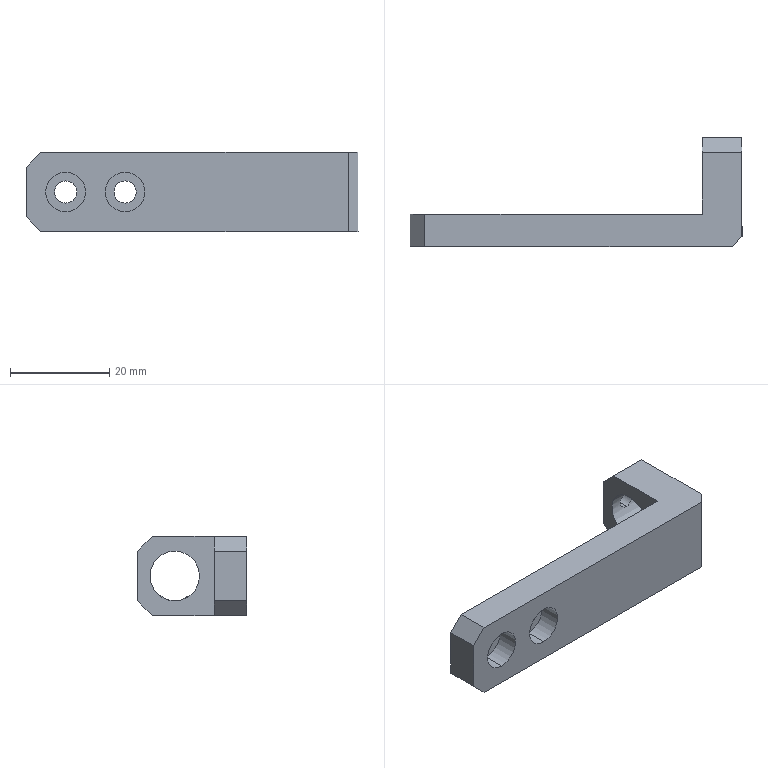Component | SolidWorks | 016WindShieldHolder-1 | 1 solid | 29 faces | box 67 x 22 x 16 mm | volume 7604 mm3 | plane 15 | cylinder 14 | commonest cylinder face diameters 3.3 x4 8 x4 4.5 x4 10 x2
build123d program:
from build123d import *

# Parameters (mm, degrees)
SKETCH1_W                                           = 67
SKETCH1_H                                           = 22
BOSS_EXTRUDE1_DEPTH                                 = 16
SKETCH2_W                                           = 59
SKETCH2_H                                           = 15.5
CUT_EXTRUDE1_DEPTH                                  = 73.312
M4_HEX_SOCKET_HEAD_CAP_SCREW_POST_HOLE1_D           = 4.5
M4_HEX_SOCKET_HEAD_CAP_SCREW_POST_HOLE1_CBORE_D     = 8
M4_HEX_SOCKET_HEAD_CAP_SCREW_POST_HOLE1_CBORE_DEPTH = 4.4
SKETCH5_R                                           = 5
CUT_EXTRUDE2_DEPTH                                  = 73.312
CHAMFER1_SIZE                                       = 3
M4_TAPPED_HOLE1_D                                   = 3.3
M4_TAPPED_HOLE1_DEPTH                               = 6.1
M4_TAPPED_HOLE1_TIP                                 = 0.9914
M4_TAPPED_HOLE2_D                                   = 3.3
M4_TAPPED_HOLE2_DEPTH                               = 6.1
M4_TAPPED_HOLE2_TIP                                 = 0.9914
CHAMFER2_SIZE                                       = 2


with BuildPart() as part:
    # Sketch1 → Boss-Extrude1 (new body)
    with BuildSketch(Plane.XY):
        with Locations((33.5, 11)):
            Rectangle(SKETCH1_W, SKETCH1_H)
    extrude(amount=BOSS_EXTRUDE1_DEPTH)

    # Sketch2 → Cut-Extrude1 (cut, through all)
    with BuildSketch(Plane.XY.offset(16)):
        with Locations((37.5, 14.25)):
            Rectangle(SKETCH2_W, SKETCH2_H)
    extrude(amount=-CUT_EXTRUDE1_DEPTH, mode=Mode.SUBTRACT)

    # M4 Hex Socket Head Cap Screw Post Hole1 (through all)
    with Locations(Plane(origin=(0, 0, 0), x_dir=(-1, 0, 0), z_dir=(0, -1, 0))):
        with Locations((-59, -8), (-47, -8)):
            CounterBoreHole(M4_HEX_SOCKET_HEAD_CAP_SCREW_POST_HOLE1_D / 2, M4_HEX_SOCKET_HEAD_CAP_SCREW_POST_HOLE1_CBORE_D / 2, M4_HEX_SOCKET_HEAD_CAP_SCREW_POST_HOLE1_CBORE_DEPTH)

    # Sketch5 → Cut-Extrude2 (cut, through all)
    with BuildSketch(Plane.ZY):
        with Locations((8, 14.5)):
            Circle(SKETCH5_R)
    extrude(amount=-CUT_EXTRUDE2_DEPTH, mode=Mode.SUBTRACT)

    # Chamfer1
    chamfer1_edges = [part.edges().sort_by_distance(p)[0] for p in [
        (67, 3.25, 16),
        (4, 22, 0),
        (4, 22, 16),
        (67, 3.25, 0),
    ]]
    chamfer(chamfer1_edges, length=CHAMFER1_SIZE)

    # M4 Tapped Hole1
    with Locations(Plane(origin=(0, 22, 0), x_dir=(1, 0, 0), z_dir=(0, 1, 0))):
        with Locations((4, -8)):
            Hole(M4_TAPPED_HOLE1_D / 2, depth=M4_TAPPED_HOLE1_DEPTH)
            with Locations((0, 0, -(M4_TAPPED_HOLE1_DEPTH + M4_TAPPED_HOLE1_TIP / 2))):  # 118° drill point
                Cone(0, M4_TAPPED_HOLE1_D / 2, M4_TAPPED_HOLE1_TIP, mode=Mode.SUBTRACT)

    # M4 Tapped Hole2
    with Locations(Plane.XY.offset(16)):
        with Locations((4, 14.5)):
            Hole(M4_TAPPED_HOLE2_D / 2, depth=M4_TAPPED_HOLE2_DEPTH)
            with Locations((0, 0, -(M4_TAPPED_HOLE2_DEPTH + M4_TAPPED_HOLE2_TIP / 2))):  # 118° drill point
                Cone(0, M4_TAPPED_HOLE2_D / 2, M4_TAPPED_HOLE2_TIP, mode=Mode.SUBTRACT)

    # Chamfer2
    chamfer2_edges = [part.edges().sort_by_distance(p)[0] for p in [
        (0, 0, 8),
    ]]
    chamfer(chamfer2_edges, length=CHAMFER2_SIZE)


solid = part.part

# Placed as in the assembly
solid = solid.moved(Location((86.76, 60.179, 19), (-180, 0, 180)))
STEP:
#1=COLOUR_RGB('',0.7922,0.8196,0.9333);
#2=FILL_AREA_STYLE_COLOUR('',#1);
#3=FILL_AREA_STYLE('',(#2));
#4=SURFACE_STYLE_FILL_AREA(#3);
#5=SURFACE_SIDE_STYLE('',(#4));
#6=SURFACE_STYLE_USAGE(.BOTH.,#5);
#7=PRESENTATION_STYLE_ASSIGNMENT((#6));
#8=CARTESIAN_POINT('',(3.323,2.94,0.2362));
#9=VERTEX_POINT('',#8);
#10=CARTESIAN_POINT('',(3.193,2.94,0.2362));
#11=VERTEX_POINT('',#10);
#12=CARTESIAN_POINT('',(3.323,2.94,0.2362));
#13=CARTESIAN_POINT('',(3.323,2.932,0.2362));
#14=CARTESIAN_POINT('',(3.321,2.923,0.2368));
#15=CARTESIAN_POINT('',(3.317,2.911,0.2383));
#16=CARTESIAN_POINT('',(3.315,2.907,0.2389));
#17=CARTESIAN_POINT('',(3.31,2.9,0.2402));
#18=CARTESIAN_POINT('',(3.307,2.897,0.2409));
#19=CARTESIAN_POINT('',(3.298,2.888,0.2431));
#20=CARTESIAN_POINT('',(3.291,2.883,0.2445));
#21=CARTESIAN_POINT('',(3.279,2.878,0.2461));
#22=CARTESIAN_POINT('',(3.275,2.877,0.2465));
#23=CARTESIAN_POINT('',(3.267,2.876,0.2471));
#24=CARTESIAN_POINT('',(3.263,2.875,0.2472));
#25=CARTESIAN_POINT('',(3.254,2.875,0.2472));
#26=CARTESIAN_POINT('',(3.25,2.876,0.2471));
#27=CARTESIAN_POINT('',(3.241,2.877,0.2465));
#28=CARTESIAN_POINT('',(3.237,2.879,0.2461));
#29=CARTESIAN_POINT('',(3.225,2.883,0.2445));
#30=CARTESIAN_POINT('',(3.218,2.888,0.2431));
#31=CARTESIAN_POINT('',(3.209,2.897,0.2409));
#32=CARTESIAN_POINT('',(3.207,2.9,0.2402));
#33=CARTESIAN_POINT('',(3.202,2.907,0.2389));
#34=CARTESIAN_POINT('',(3.2,2.911,0.2383));
#35=CARTESIAN_POINT('',(3.197,2.919,0.2373));
#36=CARTESIAN_POINT('',(3.195,2.923,0.2369));
#37=CARTESIAN_POINT('',(3.194,2.932,0.2364));
#38=CARTESIAN_POINT('',(3.193,2.936,0.2362));
#39=CARTESIAN_POINT('',(3.193,2.94,0.2362));
#40=B_SPLINE_CURVE_WITH_KNOTS('',3,(#12,#13,#14,#15,#16,#17,#18,#19,#20,#21,#22,#23,#24,#25,#26,#27,#28,#29,#30,#31,#32,#33,#34,#35,#36,#37,#38,#39),.UNSPECIFIED.,.F.,.F.,(4,2,2,2,2,2,2,2,2,2,2,2,2,4),(0.005195,0.005845,0.006169,0.006494,0.007143,0.007468,0.007792,0.008117,0.008442,0.009091,0.009415,0.00974,0.01006,0.01039),.UNSPECIFIED.);
#41=EDGE_CURVE('',#9,#11,#40,.T.);
#42=ORIENTED_EDGE('',*,*,#41,.F.);
#43=CARTESIAN_POINT('',(3.323,2.94,0.1181));
#44=VERTEX_POINT('',#43);
#45=CARTESIAN_POINT('',(3.323,2.94,0.1181));
#46=DIRECTION('',(0.,0.,-1.));
#47=VECTOR('',#46,39.37);
#48=LINE('',#45,#47);
#49=EDGE_CURVE('',#9,#44,#48,.T.);
#50=ORIENTED_EDGE('',*,*,#49,.T.);
#51=CARTESIAN_POINT('',(3.193,2.94,0.1181));
#52=VERTEX_POINT('',#51);
#53=CARTESIAN_POINT('',(3.258,2.94,0.1181));
#54=DIRECTION('',(0.,0.,-1.));
#55=DIRECTION('',(-1.,0.,-0.));
#56=AXIS2_PLACEMENT_3D('',#53,#54,#55);
#57=CIRCLE('',#56,0.06496);
#58=EDGE_CURVE('',#44,#52,#57,.T.);
#59=ORIENTED_EDGE('',*,*,#58,.T.);
#60=CARTESIAN_POINT('',(3.193,2.94,0.1181));
#61=DIRECTION('',(0.,0.,-1.));
#62=VECTOR('',#61,39.37);
#63=LINE('',#60,#62);
#64=EDGE_CURVE('',#11,#52,#63,.T.);
#65=ORIENTED_EDGE('',*,*,#64,.F.);
#66=EDGE_LOOP('',(#42,#50,#59,#65));
#67=FACE_OUTER_BOUND('',#66,.T.);
#68=CARTESIAN_POINT('',(3.258,2.94,0.1181));
#69=DIRECTION('',(0.,0.,-1.));
#70=DIRECTION('',(-1.,0.,-0.));
#71=AXIS2_PLACEMENT_3D('',#68,#69,#70);
#72=CYLINDRICAL_SURFACE('',#71,0.06496);
#73=ADVANCED_FACE('',(#67),#72,.F.);
#74=CARTESIAN_POINT('',(3.258,3.126,0.498));
#75=VERTEX_POINT('',#74);
#76=CARTESIAN_POINT('',(3.258,3.126,0.3681));
#77=VERTEX_POINT('',#76);
#78=CARTESIAN_POINT('',(3.258,3.126,0.498));
#79=CARTESIAN_POINT('',(3.267,3.126,0.498));
#80=CARTESIAN_POINT('',(3.275,3.127,0.4963));
#81=CARTESIAN_POINT('',(3.287,3.128,0.4914));
#82=CARTESIAN_POINT('',(3.291,3.129,0.4894));
#83=CARTESIAN_POINT('',(3.298,3.13,0.4847));
#84=CARTESIAN_POINT('',(3.301,3.131,0.482));
#85=CARTESIAN_POINT('',(3.31,3.133,0.473));
#86=CARTESIAN_POINT('',(3.315,3.134,0.4659));
#87=CARTESIAN_POINT('',(3.32,3.136,0.4541));
#88=CARTESIAN_POINT('',(3.321,3.136,0.45));
#89=CARTESIAN_POINT('',(3.323,3.137,0.4417));
#90=CARTESIAN_POINT('',(3.323,3.137,0.4373));
#91=CARTESIAN_POINT('',(3.323,3.137,0.4288));
#92=CARTESIAN_POINT('',(3.323,3.137,0.4245));
#93=CARTESIAN_POINT('',(3.321,3.136,0.4162));
#94=CARTESIAN_POINT('',(3.32,3.136,0.412));
#95=CARTESIAN_POINT('',(3.315,3.134,0.4003));
#96=CARTESIAN_POINT('',(3.31,3.133,0.3931));
#97=CARTESIAN_POINT('',(3.301,3.131,0.3842));
#98=CARTESIAN_POINT('',(3.298,3.13,0.3814));
#99=CARTESIAN_POINT('',(3.291,3.129,0.3767));
#100=CARTESIAN_POINT('',(3.287,3.128,0.3747));
#101=CARTESIAN_POINT('',(3.279,3.127,0.3715));
#102=CARTESIAN_POINT('',(3.275,3.127,0.3702));
#103=CARTESIAN_POINT('',(3.267,3.126,0.3685));
#104=CARTESIAN_POINT('',(3.263,3.126,0.3681));
#105=CARTESIAN_POINT('',(3.258,3.126,0.3681));
#106=B_SPLINE_CURVE_WITH_KNOTS('',3,(#78,#79,#80,#81,#82,#83,#84,#85,#86,#87,#88,#89,#90,#91,#92,#93,#94,#95,#96,#97,#98,#99,#100,#101,#102,#103,#104,#105),.UNSPECIFIED.,.F.,.F.,(4,2,2,2,2,2,2,2,2,2,2,2,2,4),(0.005195,0.005844,0.006169,0.006494,0.007143,0.007467,0.007792,0.008117,0.008441,0.009091,0.009415,0.00974,0.01006,0.01039),.UNSPECIFIED.);
#107=EDGE_CURVE('',#75,#77,#106,.T.);
#108=ORIENTED_EDGE('',*,*,#107,.F.);
#109=CARTESIAN_POINT('',(3.258,3.235,0.498));
#110=VERTEX_POINT('',#109);
#111=CARTESIAN_POINT('',(3.258,3.235,0.498));
#112=DIRECTION('',(-0.,1.,0.));
#113=VECTOR('',#112,39.37);
#114=LINE('',#111,#113);
#115=EDGE_CURVE('',#75,#110,#114,.T.);
#116=ORIENTED_EDGE('',*,*,#115,.T.);
#117=CARTESIAN_POINT('',(3.258,3.235,0.3681));
#118=VERTEX_POINT('',#117);
#119=CARTESIAN_POINT('',(3.258,3.235,0.4331));
#120=DIRECTION('',(-0.,1.,0.));
#121=DIRECTION('',(0.,0.,-1.));
#122=AXIS2_PLACEMENT_3D('',#119,#120,#121);
#123=CIRCLE('',#122,0.06496);
#124=EDGE_CURVE('',#110,#118,#123,.T.);
#125=ORIENTED_EDGE('',*,*,#124,.T.);
#126=CARTESIAN_POINT('',(3.258,3.235,0.3681));
#127=DIRECTION('',(-0.,1.,0.));
#128=VECTOR('',#127,39.37);
#129=LINE('',#126,#128);
#130=EDGE_CURVE('',#77,#118,#129,.T.);
#131=ORIENTED_EDGE('',*,*,#130,.F.);
#132=EDGE_LOOP('',(#108,#116,#125,#131));
#133=FACE_OUTER_BOUND('',#132,.T.);
#134=CARTESIAN_POINT('',(3.258,3.235,0.4331));
#135=DIRECTION('',(-0.,1.,0.));
#136=DIRECTION('',(0.,0.,-1.));
#137=AXIS2_PLACEMENT_3D('',#134,#135,#136);
#138=CYLINDRICAL_SURFACE('',#137,0.06496);
#139=ADVANCED_FACE('',(#133),#138,.F.);
#140=CARTESIAN_POINT('',(3.101,2.94,0.6299));
#141=VERTEX_POINT('',#140);
#142=CARTESIAN_POINT('',(3.101,2.94,0.2362));
#143=VERTEX_POINT('',#142);
#144=CARTESIAN_POINT('',(3.101,2.94,0.4331));
#145=DIRECTION('',(1.,0.,0.));
#146=DIRECTION('',(0.,0.,-1.));
#147=AXIS2_PLACEMENT_3D('',#144,#145,#146);
#148=CIRCLE('',#147,0.1969);
#149=EDGE_CURVE('',#141,#143,#148,.T.);
#150=ORIENTED_EDGE('',*,*,#149,.F.);
#151=CARTESIAN_POINT('',(3.416,2.94,0.6299));
#152=VERTEX_POINT('',#151);
#153=CARTESIAN_POINT('',(0.7779,2.94,0.6299));
#154=DIRECTION('',(1.,0.,0.));
#155=VECTOR('',#154,39.37);
#156=LINE('',#153,#155);
#157=EDGE_CURVE('',#141,#152,#156,.T.);
#158=ORIENTED_EDGE('',*,*,#157,.T.);
#159=CARTESIAN_POINT('',(3.416,2.94,0.2362));
#160=VERTEX_POINT('',#159);
#161=CARTESIAN_POINT('',(3.416,2.94,0.4331));
#162=DIRECTION('',(1.,0.,0.));
#163=DIRECTION('',(0.,0.,-1.));
#164=AXIS2_PLACEMENT_3D('',#161,#162,#163);
#165=CIRCLE('',#164,0.1969);
#166=EDGE_CURVE('',#152,#160,#165,.T.);
#167=ORIENTED_EDGE('',*,*,#166,.T.);
#168=CARTESIAN_POINT('',(0.7779,2.94,0.2362));
#169=DIRECTION('',(1.,0.,0.));
#170=VECTOR('',#169,39.37);
#171=LINE('',#168,#170);
#172=EDGE_CURVE('',#9,#160,#171,.T.);
#173=ORIENTED_EDGE('',*,*,#172,.F.);
#174=ORIENTED_EDGE('',*,*,#41,.T.);
#175=CARTESIAN_POINT('',(0.7779,2.94,0.2362));
#176=DIRECTION('',(1.,0.,0.));
#177=VECTOR('',#176,39.37);
#178=LINE('',#175,#177);
#179=EDGE_CURVE('',#143,#11,#178,.T.);
#180=ORIENTED_EDGE('',*,*,#179,.F.);
#181=EDGE_LOOP('',(#150,#158,#167,#173,#174,#180));
#182=FACE_OUTER_BOUND('',#181,.T.);
#183=CARTESIAN_POINT('',(0.7779,2.94,0.4331));
#184=DIRECTION('',(1.,0.,0.));
#185=DIRECTION('',(0.,0.,-1.));
#186=AXIS2_PLACEMENT_3D('',#183,#184,#185);
#187=CYLINDRICAL_SURFACE('',#186,0.1969);
#188=ADVANCED_FACE('',(#182),#187,.F.);
#189=CARTESIAN_POINT('',(1.093,2.542,0.2756));
#190=VERTEX_POINT('',#189);
#191=CARTESIAN_POINT('',(1.093,2.542,0.5906));
#192=VERTEX_POINT('',#191);
#193=CARTESIAN_POINT('',(1.093,2.542,0.4331));
#194=DIRECTION('',(0.,-1.,-0.));
#195=DIRECTION('',(-0.,0.,1.));
#196=AXIS2_PLACEMENT_3D('',#193,#194,#195);
#197=CIRCLE('',#196,0.1575);
#198=EDGE_CURVE('',#190,#192,#197,.T.);
#199=ORIENTED_EDGE('',*,*,#198,.F.);
#200=CARTESIAN_POINT('',(1.093,2.369,0.2756));
#201=VERTEX_POINT('',#200);
#202=CARTESIAN_POINT('',(1.093,2.369,0.2756));
#203=DIRECTION('',(0.,-1.,-0.));
#204=VECTOR('',#203,39.37);
#205=LINE('',#202,#204);
#206=EDGE_CURVE('',#190,#201,#205,.T.);
#207=ORIENTED_EDGE('',*,*,#206,.T.);
#208=CARTESIAN_POINT('',(1.093,2.369,0.5906));
#209=VERTEX_POINT('',#208);
#210=CARTESIAN_POINT('',(1.093,2.369,0.4331));
#211=DIRECTION('',(0.,-1.,-0.));
#212=DIRECTION('',(-0.,0.,1.));
#213=AXIS2_PLACEMENT_3D('',#210,#211,#212);
#214=CIRCLE('',#213,0.1575);
#215=EDGE_CURVE('',#201,#209,#214,.T.);
#216=ORIENTED_EDGE('',*,*,#215,.T.);
#217=CARTESIAN_POINT('',(1.093,2.369,0.5906));
#218=DIRECTION('',(0.,-1.,-0.));
#219=VECTOR('',#218,39.37);
#220=LINE('',#217,#219);
#221=EDGE_CURVE('',#192,#209,#220,.T.);
#222=ORIENTED_EDGE('',*,*,#221,.F.);
#223=EDGE_LOOP('',(#199,#207,#216,#222));
#224=FACE_OUTER_BOUND('',#223,.T.);
#225=CARTESIAN_POINT('',(1.093,2.369,0.4331));
#226=DIRECTION('',(0.,-1.,-0.));
#227=DIRECTION('',(-0.,0.,1.));
#228=AXIS2_PLACEMENT_3D('',#225,#226,#227);
#229=CYLINDRICAL_SURFACE('',#228,0.1575);
#230=ADVANCED_FACE('',(#224),#229,.F.);
#231=CARTESIAN_POINT('',(1.093,2.625,0.3445));
#232=VERTEX_POINT('',#231);
#233=CARTESIAN_POINT('',(1.093,2.625,0.5217));
#234=VERTEX_POINT('',#233);
#235=CARTESIAN_POINT('',(1.093,2.625,0.4331));
#236=DIRECTION('',(0.,-1.,-0.));
#237=DIRECTION('',(-1.,0.,-0.));
#238=AXIS2_PLACEMENT_3D('',#235,#236,#237);
#239=CIRCLE('',#238,0.08858);
#240=EDGE_CURVE('',#232,#234,#239,.T.);
#241=ORIENTED_EDGE('',*,*,#240,.F.);
#242=CARTESIAN_POINT('',(1.093,2.542,0.3445));
#243=VERTEX_POINT('',#242);
#244=CARTESIAN_POINT('',(1.093,2.369,0.3445));
#245=DIRECTION('',(0.,-1.,-0.));
#246=VECTOR('',#245,39.37);
#247=LINE('',#244,#246);
#248=EDGE_CURVE('',#232,#243,#247,.T.);
#249=ORIENTED_EDGE('',*,*,#248,.T.);
#250=CARTESIAN_POINT('',(1.093,2.542,0.5217));
#251=VERTEX_POINT('',#250);
#252=CARTESIAN_POINT('',(1.093,2.542,0.4331));
#253=DIRECTION('',(0.,-1.,-0.));
#254=DIRECTION('',(-0.,0.,1.));
#255=AXIS2_PLACEMENT_3D('',#252,#253,#254);
#256=CIRCLE('',#255,0.08858);
#257=EDGE_CURVE('',#243,#251,#256,.T.);
#258=ORIENTED_EDGE('',*,*,#257,.T.);
#259=CARTESIAN_POINT('',(1.093,2.369,0.5217));
#260=DIRECTION('',(0.,-1.,-0.));
#261=VECTOR('',#260,39.37);
#262=LINE('',#259,#261);
#263=EDGE_CURVE('',#234,#251,#262,.T.);
#264=ORIENTED_EDGE('',*,*,#263,.F.);
#265=EDGE_LOOP('',(#241,#249,#258,#264));
#266=FACE_OUTER_BOUND('',#265,.T.);
#267=CARTESIAN_POINT('',(1.093,2.369,0.4331));
#268=DIRECTION('',(0.,-1.,-0.));
#269=DIRECTION('',(-0.,0.,1.));
#270=AXIS2_PLACEMENT_3D('',#267,#268,#269);
#271=CYLINDRICAL_SURFACE('',#270,0.08858);
#272=ADVANCED_FACE('',(#266),#271,.F.);
#273=CARTESIAN_POINT('',(1.565,2.542,0.2756));
#274=VERTEX_POINT('',#273);
#275=CARTESIAN_POINT('',(1.565,2.542,0.5906));
#276=VERTEX_POINT('',#275);
#277=CARTESIAN_POINT('',(1.565,2.542,0.4331));
#278=DIRECTION('',(0.,-1.,-0.));
#279=DIRECTION('',(-0.,0.,1.));
#280=AXIS2_PLACEMENT_3D('',#277,#278,#279);
#281=CIRCLE('',#280,0.1575);
#282=EDGE_CURVE('',#274,#276,#281,.T.);
#283=ORIENTED_EDGE('',*,*,#282,.F.);
#284=CARTESIAN_POINT('',(1.565,2.369,0.2756));
#285=VERTEX_POINT('',#284);
#286=CARTESIAN_POINT('',(1.565,2.369,0.2756));
#287=DIRECTION('',(0.,-1.,-0.));
#288=VECTOR('',#287,39.37);
#289=LINE('',#286,#288);
#290=EDGE_CURVE('',#274,#285,#289,.T.);
#291=ORIENTED_EDGE('',*,*,#290,.T.);
#292=CARTESIAN_POINT('',(1.565,2.369,0.5906));
#293=VERTEX_POINT('',#292);
#294=CARTESIAN_POINT('',(1.565,2.369,0.4331));
#295=DIRECTION('',(0.,-1.,-0.));
#296=DIRECTION('',(-0.,0.,1.));
#297=AXIS2_PLACEMENT_3D('',#294,#295,#296);
#298=CIRCLE('',#297,0.1575);
#299=EDGE_CURVE('',#285,#293,#298,.T.);
#300=ORIENTED_EDGE('',*,*,#299,.T.);
#301=CARTESIAN_POINT('',(1.565,2.369,0.5906));
#302=DIRECTION('',(0.,-1.,-0.));
#303=VECTOR('',#302,39.37);
#304=LINE('',#301,#303);
#305=EDGE_CURVE('',#276,#293,#304,.T.);
#306=ORIENTED_EDGE('',*,*,#305,.F.);
#307=EDGE_LOOP('',(#283,#291,#300,#306));
#308=FACE_OUTER_BOUND('',#307,.T.);
#309=CARTESIAN_POINT('',(1.565,2.369,0.4331));
#310=DIRECTION('',(0.,-1.,-0.));
#311=DIRECTION('',(-0.,0.,1.));
#312=AXIS2_PLACEMENT_3D('',#309,#310,#311);
#313=CYLINDRICAL_SURFACE('',#312,0.1575);
#314=ADVANCED_FACE('',(#308),#313,.F.);
#315=CARTESIAN_POINT('',(1.565,2.625,0.3445));
#316=VERTEX_POINT('',#315);
#317=CARTESIAN_POINT('',(1.565,2.625,0.5217));
#318=VERTEX_POINT('',#317);
#319=CARTESIAN_POINT('',(1.565,2.625,0.4331));
#320=DIRECTION('',(0.,-1.,-0.));
#321=DIRECTION('',(-1.,0.,-0.));
#322=AXIS2_PLACEMENT_3D('',#319,#320,#321);
#323=CIRCLE('',#322,0.08858);
#324=EDGE_CURVE('',#316,#318,#323,.T.);
#325=ORIENTED_EDGE('',*,*,#324,.F.);
#326=CARTESIAN_POINT('',(1.565,2.542,0.3445));
#327=VERTEX_POINT('',#326);
#328=CARTESIAN_POINT('',(1.565,2.369,0.3445));
#329=DIRECTION('',(0.,-1.,-0.));
#330=VECTOR('',#329,39.37);
#331=LINE('',#328,#330);
#332=EDGE_CURVE('',#316,#327,#331,.T.);
#333=ORIENTED_EDGE('',*,*,#332,.T.);
#334=CARTESIAN_POINT('',(1.565,2.542,0.5217));
#335=VERTEX_POINT('',#334);
#336=CARTESIAN_POINT('',(1.565,2.542,0.4331));
#337=DIRECTION('',(0.,-1.,-0.));
#338=DIRECTION('',(-0.,0.,1.));
#339=AXIS2_PLACEMENT_3D('',#336,#337,#338);
#340=CIRCLE('',#339,0.08858);
#341=EDGE_CURVE('',#327,#335,#340,.T.);
#342=ORIENTED_EDGE('',*,*,#341,.T.);
#343=CARTESIAN_POINT('',(1.565,2.369,0.5217));
#344=DIRECTION('',(0.,-1.,-0.));
#345=VECTOR('',#344,39.37);
#346=LINE('',#343,#345);
#347=EDGE_CURVE('',#318,#335,#346,.T.);
#348=ORIENTED_EDGE('',*,*,#347,.F.);
#349=EDGE_LOOP('',(#325,#333,#342,#348));
#350=FACE_OUTER_BOUND('',#349,.T.);
#351=CARTESIAN_POINT('',(1.565,2.369,0.4331));
#352=DIRECTION('',(0.,-1.,-0.));
#353=DIRECTION('',(-0.,0.,1.));
#354=AXIS2_PLACEMENT_3D('',#351,#352,#353);
#355=CYLINDRICAL_SURFACE('',#354,0.08858);
#356=ADVANCED_FACE('',(#350),#355,.F.);
#357=CARTESIAN_POINT('',(3.416,2.94,0.4331));
#358=DIRECTION('',(1.,0.,0.));
#359=DIRECTION('',(0.,0.,-1.));
#360=AXIS2_PLACEMENT_3D('',#357,#358,#359);
#361=CIRCLE('',#360,0.1969);
#362=EDGE_CURVE('',#160,#152,#361,.T.);
#363=ORIENTED_EDGE('',*,*,#362,.F.);
#364=ORIENTED_EDGE('',*,*,#166,.F.);
#365=EDGE_LOOP('',(#363,#364));
#366=FACE_BOUND('',#365,.T.);
#367=CARTESIAN_POINT('',(3.416,3.117,0.748));
#368=VERTEX_POINT('',#367);
#369=CARTESIAN_POINT('',(3.416,2.448,0.748));
#370=VERTEX_POINT('',#369);
#371=CARTESIAN_POINT('',(3.416,2.369,0.748));
#372=DIRECTION('',(0.,-1.,-0.));
#373=VECTOR('',#372,39.37);
#374=LINE('',#371,#373);
#375=EDGE_CURVE('',#368,#370,#374,.T.);
#376=ORIENTED_EDGE('',*,*,#375,.T.);
#377=CARTESIAN_POINT('',(3.416,2.448,0.1181));
#378=VERTEX_POINT('',#377);
#379=CARTESIAN_POINT('',(3.416,2.448,0.1181));
#380=DIRECTION('',(0.,0.,-1.));
#381=VECTOR('',#380,39.37);
#382=LINE('',#379,#381);
#383=EDGE_CURVE('',#370,#378,#382,.T.);
#384=ORIENTED_EDGE('',*,*,#383,.T.);
#385=CARTESIAN_POINT('',(3.416,3.117,0.1181));
#386=VERTEX_POINT('',#385);
#387=CARTESIAN_POINT('',(3.416,2.369,0.1181));
#388=DIRECTION('',(0.,-1.,-0.));
#389=VECTOR('',#388,39.37);
#390=LINE('',#387,#389);
#391=EDGE_CURVE('',#386,#378,#390,.T.);
#392=ORIENTED_EDGE('',*,*,#391,.F.);
#393=CARTESIAN_POINT('',(3.416,3.235,0.2362));
#394=VERTEX_POINT('',#393);
#395=CARTESIAN_POINT('',(3.416,3.117,0.1181));
#396=DIRECTION('',(-0.,0.7071,0.7071));
#397=VECTOR('',#396,39.37);
#398=LINE('',#395,#397);
#399=EDGE_CURVE('',#386,#394,#398,.T.);
#400=ORIENTED_EDGE('',*,*,#399,.T.);
#401=CARTESIAN_POINT('',(3.416,3.235,0.6299));
#402=VERTEX_POINT('',#401);
#403=CARTESIAN_POINT('',(3.416,3.235,0.1181));
#404=DIRECTION('',(-0.,-0.,1.));
#405=VECTOR('',#404,39.37);
#406=LINE('',#403,#405);
#407=EDGE_CURVE('',#394,#402,#406,.T.);
#408=ORIENTED_EDGE('',*,*,#407,.T.);
#409=CARTESIAN_POINT('',(3.416,3.235,0.6299));
#410=DIRECTION('',(-0.,-0.7071,0.7071));
#411=VECTOR('',#410,39.37);
#412=LINE('',#409,#411);
#413=EDGE_CURVE('',#402,#368,#412,.T.);
#414=ORIENTED_EDGE('',*,*,#413,.T.);
#415=EDGE_LOOP('',(#376,#384,#392,#400,#408,#414));
#416=FACE_OUTER_BOUND('',#415,.T.);
#417=CARTESIAN_POINT('',(3.416,2.369,0.1181));
#418=DIRECTION('',(-1.,-0.,-0.));
#419=DIRECTION('',(-0.,-0.,1.));
#420=AXIS2_PLACEMENT_3D('',#417,#418,#419);
#421=PLANE('',#420);
#422=ADVANCED_FACE('',(#366,#416),#421,.F.);
#423=CARTESIAN_POINT('',(1.093,2.369,0.4331));
#424=DIRECTION('',(0.,-1.,-0.));
#425=DIRECTION('',(-0.,0.,1.));
#426=AXIS2_PLACEMENT_3D('',#423,#424,#425);
#427=CIRCLE('',#426,0.1575);
#428=EDGE_CURVE('',#209,#201,#427,.T.);
#429=ORIENTED_EDGE('',*,*,#428,.F.);
#430=ORIENTED_EDGE('',*,*,#215,.F.);
#431=EDGE_LOOP('',(#429,#430));
#432=FACE_BOUND('',#431,.T.);
#433=CARTESIAN_POINT('',(1.565,2.369,0.4331));
#434=DIRECTION('',(0.,-1.,-0.));
#435=DIRECTION('',(-0.,0.,1.));
#436=AXIS2_PLACEMENT_3D('',#433,#434,#435);
#437=CIRCLE('',#436,0.1575);
#438=EDGE_CURVE('',#293,#285,#437,.T.);
#439=ORIENTED_EDGE('',*,*,#438,.F.);
#440=ORIENTED_EDGE('',*,*,#299,.F.);
#441=EDGE_LOOP('',(#439,#440));
#442=FACE_BOUND('',#441,.T.);
#443=CARTESIAN_POINT('',(3.337,2.369,0.1181));
#444=VERTEX_POINT('',#443);
#445=CARTESIAN_POINT('',(0.8961,2.369,0.1181));
#446=VERTEX_POINT('',#445);
#447=CARTESIAN_POINT('',(3.416,2.369,0.1181));
#448=DIRECTION('',(-1.,-0.,-0.));
#449=VECTOR('',#448,39.37);
#450=LINE('',#447,#449);
#451=EDGE_CURVE('',#444,#446,#450,.T.);
#452=ORIENTED_EDGE('',*,*,#451,.F.);
#453=CARTESIAN_POINT('',(3.337,2.369,0.748));
#454=VERTEX_POINT('',#453);
#455=CARTESIAN_POINT('',(3.337,2.369,0.1181));
#456=DIRECTION('',(-0.,-0.,1.));
#457=VECTOR('',#456,39.37);
#458=LINE('',#455,#457);
#459=EDGE_CURVE('',#444,#454,#458,.T.);
#460=ORIENTED_EDGE('',*,*,#459,.T.);
#461=CARTESIAN_POINT('',(0.8961,2.369,0.748));
#462=VERTEX_POINT('',#461);
#463=CARTESIAN_POINT('',(3.416,2.369,0.748));
#464=DIRECTION('',(-1.,-0.,-0.));
#465=VECTOR('',#464,39.37);
#466=LINE('',#463,#465);
#467=EDGE_CURVE('',#454,#462,#466,.T.);
#468=ORIENTED_EDGE('',*,*,#467,.T.);
#469=CARTESIAN_POINT('',(0.7779,2.369,0.6299));
#470=VERTEX_POINT('',#469);
#471=CARTESIAN_POINT('',(0.7779,2.369,0.6299));
#472=DIRECTION('',(-0.7071,-0.,-0.7071));
#473=VECTOR('',#472,39.37);
#474=LINE('',#471,#473);
#475=EDGE_CURVE('',#462,#470,#474,.T.);
#476=ORIENTED_EDGE('',*,*,#475,.T.);
#477=CARTESIAN_POINT('',(0.7779,2.369,0.2362));
#478=VERTEX_POINT('',#477);
#479=CARTESIAN_POINT('',(0.7779,2.369,0.1181));
#480=DIRECTION('',(-0.,-0.,1.));
#481=VECTOR('',#480,39.37);
#482=LINE('',#479,#481);
#483=EDGE_CURVE('',#478,#470,#482,.T.);
#484=ORIENTED_EDGE('',*,*,#483,.F.);
#485=CARTESIAN_POINT('',(0.8961,2.369,0.1181));
#486=DIRECTION('',(0.7071,0.,-0.7071));
#487=VECTOR('',#486,39.37);
#488=LINE('',#485,#487);
#489=EDGE_CURVE('',#478,#446,#488,.T.);
#490=ORIENTED_EDGE('',*,*,#489,.T.);
#491=EDGE_LOOP('',(#452,#460,#468,#476,#484,#490));
#492=FACE_OUTER_BOUND('',#491,.T.);
#493=CARTESIAN_POINT('',(3.416,2.369,0.1181));
#494=DIRECTION('',(-0.,1.,0.));
#495=DIRECTION('',(0.,0.,-1.));
#496=AXIS2_PLACEMENT_3D('',#493,#494,#495);
#497=PLANE('',#496);
#498=ADVANCED_FACE('',(#432,#442,#492),#497,.F.);
#499=ORIENTED_EDGE('',*,*,#483,.T.);
#500=CARTESIAN_POINT('',(0.7779,2.625,0.6299));
#501=VERTEX_POINT('',#500);
#502=CARTESIAN_POINT('',(0.7779,2.625,0.6299));
#503=DIRECTION('',(-0.,1.,0.));
#504=VECTOR('',#503,39.37);
#505=LINE('',#502,#504);
#506=EDGE_CURVE('',#470,#501,#505,.T.);
#507=ORIENTED_EDGE('',*,*,#506,.T.);
#508=CARTESIAN_POINT('',(0.7779,2.625,0.2362));
#509=VERTEX_POINT('',#508);
#510=CARTESIAN_POINT('',(0.7779,2.625,0.748));
#511=DIRECTION('',(0.,0.,-1.));
#512=VECTOR('',#511,39.37);
#513=LINE('',#510,#512);
#514=EDGE_CURVE('',#501,#509,#513,.T.);
#515=ORIENTED_EDGE('',*,*,#514,.T.);
#516=CARTESIAN_POINT('',(0.7779,2.369,0.2362));
#517=DIRECTION('',(0.,-1.,-0.));
#518=VECTOR('',#517,39.37);
#519=LINE('',#516,#518);
#520=EDGE_CURVE('',#509,#478,#519,.T.);
#521=ORIENTED_EDGE('',*,*,#520,.T.);
#522=EDGE_LOOP('',(#499,#507,#515,#521));
#523=FACE_OUTER_BOUND('',#522,.T.);
#524=CARTESIAN_POINT('',(0.7779,2.369,0.1181));
#525=DIRECTION('',(1.,0.,0.));
#526=DIRECTION('',(0.,0.,-1.));
#527=AXIS2_PLACEMENT_3D('',#524,#525,#526);
#528=PLANE('',#527);
#529=ADVANCED_FACE('',(#523),#528,.F.);
#530=CARTESIAN_POINT('',(3.258,3.235,0.4331));
#531=DIRECTION('',(-0.,1.,0.));
#532=DIRECTION('',(0.,0.,-1.));
#533=AXIS2_PLACEMENT_3D('',#530,#531,#532);
#534=CIRCLE('',#533,0.06496);
#535=EDGE_CURVE('',#118,#110,#534,.T.);
#536=ORIENTED_EDGE('',*,*,#535,.F.);
#537=ORIENTED_EDGE('',*,*,#124,.F.);
#538=EDGE_LOOP('',(#536,#537));
#539=FACE_BOUND('',#538,.T.);
#540=CARTESIAN_POINT('',(3.101,3.235,0.6299));
#541=VERTEX_POINT('',#540);
#542=CARTESIAN_POINT('',(3.101,3.235,0.2362));
#543=VERTEX_POINT('',#542);
#544=CARTESIAN_POINT('',(3.101,3.235,0.748));
#545=DIRECTION('',(0.,0.,-1.));
#546=VECTOR('',#545,39.37);
#547=LINE('',#544,#546);
#548=EDGE_CURVE('',#541,#543,#547,.T.);
#549=ORIENTED_EDGE('',*,*,#548,.F.);
#550=CARTESIAN_POINT('',(3.416,3.235,0.6299));
#551=DIRECTION('',(1.,0.,0.));
#552=VECTOR('',#551,39.37);
#553=LINE('',#550,#552);
#554=EDGE_CURVE('',#541,#402,#553,.T.);
#555=ORIENTED_EDGE('',*,*,#554,.T.);
#556=ORIENTED_EDGE('',*,*,#407,.F.);
#557=CARTESIAN_POINT('',(3.416,3.235,0.2362));
#558=DIRECTION('',(-1.,-0.,-0.));
#559=VECTOR('',#558,39.37);
#560=LINE('',#557,#559);
#561=EDGE_CURVE('',#394,#543,#560,.T.);
#562=ORIENTED_EDGE('',*,*,#561,.T.);
#563=EDGE_LOOP('',(#549,#555,#556,#562));
#564=FACE_OUTER_BOUND('',#563,.T.);
#565=CARTESIAN_POINT('',(3.416,3.235,0.1181));
#566=DIRECTION('',(0.,-1.,-0.));
#567=DIRECTION('',(-0.,-0.,1.));
#568=AXIS2_PLACEMENT_3D('',#565,#566,#567);
#569=PLANE('',#568);
#570=ADVANCED_FACE('',(#539,#564),#569,.F.);
#571=CARTESIAN_POINT('',(3.258,2.94,0.1181));
#572=DIRECTION('',(0.,0.,-1.));
#573=DIRECTION('',(-1.,0.,-0.));
#574=AXIS2_PLACEMENT_3D('',#571,#572,#573);
#575=CIRCLE('',#574,0.06496);
#576=EDGE_CURVE('',#52,#44,#575,.T.);
#577=ORIENTED_EDGE('',*,*,#576,.F.);
#578=ORIENTED_EDGE('',*,*,#58,.F.);
#579=EDGE_LOOP('',(#577,#578));
#580=FACE_BOUND('',#579,.T.);
#581=ORIENTED_EDGE('',*,*,#391,.T.);
#582=CARTESIAN_POINT('',(3.337,2.369,0.1181));
#583=DIRECTION('',(-0.7071,-0.7071,-0.));
#584=VECTOR('',#583,39.37);
#585=LINE('',#582,#584);
#586=EDGE_CURVE('',#378,#444,#585,.T.);
#587=ORIENTED_EDGE('',*,*,#586,.T.);
#588=ORIENTED_EDGE('',*,*,#451,.T.);
#589=CARTESIAN_POINT('',(0.8961,2.625,0.1181));
#590=VERTEX_POINT('',#589);
#591=CARTESIAN_POINT('',(0.8961,2.369,0.1181));
#592=DIRECTION('',(-0.,1.,0.));
#593=VECTOR('',#592,39.37);
#594=LINE('',#591,#593);
#595=EDGE_CURVE('',#446,#590,#594,.T.);
#596=ORIENTED_EDGE('',*,*,#595,.T.);
#597=CARTESIAN_POINT('',(3.101,2.625,0.1181));
#598=VERTEX_POINT('',#597);
#599=CARTESIAN_POINT('',(0.7779,2.625,0.1181));
#600=DIRECTION('',(-1.,-0.,-0.));
#601=VECTOR('',#600,39.37);
#602=LINE('',#599,#601);
#603=EDGE_CURVE('',#598,#590,#602,.T.);
#604=ORIENTED_EDGE('',*,*,#603,.F.);
#605=CARTESIAN_POINT('',(3.101,3.117,0.1181));
#606=VERTEX_POINT('',#605);
#607=CARTESIAN_POINT('',(3.101,3.235,0.1181));
#608=DIRECTION('',(0.,-1.,-0.));
#609=VECTOR('',#608,39.37);
#610=LINE('',#607,#609);
#611=EDGE_CURVE('',#606,#598,#610,.T.);
#612=ORIENTED_EDGE('',*,*,#611,.F.);
#613=CARTESIAN_POINT('',(3.416,3.117,0.1181));
#614=DIRECTION('',(1.,0.,0.));
#615=VECTOR('',#614,39.37);
#616=LINE('',#613,#615);
#617=EDGE_CURVE('',#606,#386,#616,.T.);
#618=ORIENTED_EDGE('',*,*,#617,.T.);
#619=EDGE_LOOP('',(#581,#587,#588,#596,#604,#612,#618));
#620=FACE_OUTER_BOUND('',#619,.T.);
#621=CARTESIAN_POINT('',(3.416,2.369,0.1181));
#622=DIRECTION('',(-0.,-0.,1.));
#623=DIRECTION('',(1.,0.,0.));
#624=AXIS2_PLACEMENT_3D('',#621,#622,#623);
#625=PLANE('',#624);
#626=ADVANCED_FACE('',(#580,#620),#625,.F.);
#627=ORIENTED_EDGE('',*,*,#467,.F.);
#628=CARTESIAN_POINT('',(3.376,2.409,0.748));
#629=DIRECTION('',(0.7071,0.7071,0.));
#630=VECTOR('',#629,39.37);
#631=LINE('',#628,#630);
#632=EDGE_CURVE('',#454,#370,#631,.T.);
#633=ORIENTED_EDGE('',*,*,#632,.T.);
#634=ORIENTED_EDGE('',*,*,#375,.F.);
#635=CARTESIAN_POINT('',(3.101,3.117,0.748));
#636=VERTEX_POINT('',#635);
#637=CARTESIAN_POINT('',(3.101,3.117,0.748));
#638=DIRECTION('',(-1.,-0.,-0.));
#639=VECTOR('',#638,39.37);
#640=LINE('',#637,#639);
#641=EDGE_CURVE('',#368,#636,#640,.T.);
#642=ORIENTED_EDGE('',*,*,#641,.T.);
#643=CARTESIAN_POINT('',(3.101,2.625,0.748));
#644=VERTEX_POINT('',#643);
#645=CARTESIAN_POINT('',(3.101,3.235,0.748));
#646=DIRECTION('',(0.,-1.,-0.));
#647=VECTOR('',#646,39.37);
#648=LINE('',#645,#647);
#649=EDGE_CURVE('',#636,#644,#648,.T.);
#650=ORIENTED_EDGE('',*,*,#649,.T.);
#651=CARTESIAN_POINT('',(0.8961,2.625,0.748));
#652=VERTEX_POINT('',#651);
#653=CARTESIAN_POINT('',(0.7779,2.625,0.748));
#654=DIRECTION('',(-1.,-0.,-0.));
#655=VECTOR('',#654,39.37);
#656=LINE('',#653,#655);
#657=EDGE_CURVE('',#644,#652,#656,.T.);
#658=ORIENTED_EDGE('',*,*,#657,.T.);
#659=CARTESIAN_POINT('',(0.8961,2.369,0.748));
#660=DIRECTION('',(0.,-1.,-0.));
#661=VECTOR('',#660,39.37);
#662=LINE('',#659,#661);
#663=EDGE_CURVE('',#652,#462,#662,.T.);
#664=ORIENTED_EDGE('',*,*,#663,.T.);
#665=EDGE_LOOP('',(#627,#633,#634,#642,#650,#658,#664));
#666=FACE_OUTER_BOUND('',#665,.T.);
#667=CARTESIAN_POINT('',(3.416,2.369,0.748));
#668=DIRECTION('',(-0.,-0.,1.));
#669=DIRECTION('',(1.,0.,0.));
#670=AXIS2_PLACEMENT_3D('',#667,#668,#669);
#671=PLANE('',#670);
#672=ADVANCED_FACE('',(#666),#671,.T.);
#673=CARTESIAN_POINT('',(1.093,2.625,0.4331));
#674=DIRECTION('',(0.,-1.,-0.));
#675=DIRECTION('',(-1.,0.,-0.));
#676=AXIS2_PLACEMENT_3D('',#673,#674,#675);
#677=CIRCLE('',#676,0.08858);
#678=EDGE_CURVE('',#234,#232,#677,.T.);
#679=ORIENTED_EDGE('',*,*,#678,.T.);
#680=ORIENTED_EDGE('',*,*,#240,.T.);
#681=EDGE_LOOP('',(#679,#680));
#682=FACE_BOUND('',#681,.T.);
#683=CARTESIAN_POINT('',(1.565,2.625,0.4331));
#684=DIRECTION('',(0.,-1.,-0.));
#685=DIRECTION('',(-1.,0.,-0.));
#686=AXIS2_PLACEMENT_3D('',#683,#684,#685);
#687=CIRCLE('',#686,0.08858);
#688=EDGE_CURVE('',#318,#316,#687,.T.);
#689=ORIENTED_EDGE('',*,*,#688,.T.);
#690=ORIENTED_EDGE('',*,*,#324,.T.);
#691=EDGE_LOOP('',(#689,#690));
#692=FACE_BOUND('',#691,.T.);
#693=ORIENTED_EDGE('',*,*,#514,.F.);
#694=CARTESIAN_POINT('',(0.7779,2.625,0.6299));
#695=DIRECTION('',(0.7071,0.,0.7071));
#696=VECTOR('',#695,39.37);
#697=LINE('',#694,#696);
#698=EDGE_CURVE('',#501,#652,#697,.T.);
#699=ORIENTED_EDGE('',*,*,#698,.T.);
#700=ORIENTED_EDGE('',*,*,#657,.F.);
#701=CARTESIAN_POINT('',(3.101,2.625,0.748));
#702=DIRECTION('',(0.,0.,-1.));
#703=VECTOR('',#702,39.37);
#704=LINE('',#701,#703);
#705=EDGE_CURVE('',#644,#598,#704,.T.);
#706=ORIENTED_EDGE('',*,*,#705,.T.);
#707=ORIENTED_EDGE('',*,*,#603,.T.);
#708=CARTESIAN_POINT('',(0.8961,2.625,0.1181));
#709=DIRECTION('',(-0.7071,-0.,0.7071));
#710=VECTOR('',#709,39.37);
#711=LINE('',#708,#710);
#712=EDGE_CURVE('',#590,#509,#711,.T.);
#713=ORIENTED_EDGE('',*,*,#712,.T.);
#714=EDGE_LOOP('',(#693,#699,#700,#706,#707,#713));
#715=FACE_OUTER_BOUND('',#714,.T.);
#716=CARTESIAN_POINT('',(0.7779,2.625,0.748));
#717=DIRECTION('',(0.,-1.,-0.));
#718=DIRECTION('',(-1.,-0.,-0.));
#719=AXIS2_PLACEMENT_3D('',#716,#717,#718);
#720=PLANE('',#719);
#721=ADVANCED_FACE('',(#682,#692,#715),#720,.F.);
#722=CARTESIAN_POINT('',(3.101,2.94,0.4331));
#723=DIRECTION('',(1.,0.,0.));
#724=DIRECTION('',(0.,0.,-1.));
#725=AXIS2_PLACEMENT_3D('',#722,#723,#724);
#726=CIRCLE('',#725,0.1969);
#727=EDGE_CURVE('',#143,#141,#726,.T.);
#728=ORIENTED_EDGE('',*,*,#727,.T.);
#729=ORIENTED_EDGE('',*,*,#149,.T.);
#730=EDGE_LOOP('',(#728,#729));
#731=FACE_BOUND('',#730,.T.);
#732=ORIENTED_EDGE('',*,*,#649,.F.);
#733=CARTESIAN_POINT('',(3.101,3.235,0.6299));
#734=DIRECTION('',(0.,0.7071,-0.7071));
#735=VECTOR('',#734,39.37);
#736=LINE('',#733,#735);
#737=EDGE_CURVE('',#636,#541,#736,.T.);
#738=ORIENTED_EDGE('',*,*,#737,.T.);
#739=ORIENTED_EDGE('',*,*,#548,.T.);
#740=CARTESIAN_POINT('',(3.101,3.117,0.1181));
#741=DIRECTION('',(0.,-0.7071,-0.7071));
#742=VECTOR('',#741,39.37);
#743=LINE('',#740,#742);
#744=EDGE_CURVE('',#543,#606,#743,.T.);
#745=ORIENTED_EDGE('',*,*,#744,.T.);
#746=ORIENTED_EDGE('',*,*,#611,.T.);
#747=ORIENTED_EDGE('',*,*,#705,.F.);
#748=EDGE_LOOP('',(#732,#738,#739,#745,#746,#747));
#749=FACE_OUTER_BOUND('',#748,.T.);
#750=CARTESIAN_POINT('',(3.101,3.235,0.748));
#751=DIRECTION('',(1.,0.,0.));
#752=DIRECTION('',(0.,0.,-1.));
#753=AXIS2_PLACEMENT_3D('',#750,#751,#752);
#754=PLANE('',#753);
#755=ADVANCED_FACE('',(#731,#749),#754,.F.);
#756=ORIENTED_EDGE('',*,*,#332,.F.);
#757=ORIENTED_EDGE('',*,*,#688,.F.);
#758=ORIENTED_EDGE('',*,*,#347,.T.);
#759=CARTESIAN_POINT('',(1.565,2.542,0.4331));
#760=DIRECTION('',(0.,-1.,-0.));
#761=DIRECTION('',(-0.,0.,1.));
#762=AXIS2_PLACEMENT_3D('',#759,#760,#761);
#763=CIRCLE('',#762,0.08858);
#764=EDGE_CURVE('',#335,#327,#763,.T.);
#765=ORIENTED_EDGE('',*,*,#764,.T.);
#766=EDGE_LOOP('',(#756,#757,#758,#765));
#767=FACE_OUTER_BOUND('',#766,.T.);
#768=CARTESIAN_POINT('',(1.565,2.369,0.4331));
#769=DIRECTION('',(0.,-1.,-0.));
#770=DIRECTION('',(-0.,0.,1.));
#771=AXIS2_PLACEMENT_3D('',#768,#769,#770);
#772=CYLINDRICAL_SURFACE('',#771,0.08858);
#773=ADVANCED_FACE('',(#767),#772,.F.);
#774=ORIENTED_EDGE('',*,*,#764,.F.);
#775=ORIENTED_EDGE('',*,*,#341,.F.);
#776=EDGE_LOOP('',(#774,#775));
#777=FACE_BOUND('',#776,.T.);
#778=CARTESIAN_POINT('',(1.565,2.542,0.4331));
#779=DIRECTION('',(0.,-1.,-0.));
#780=DIRECTION('',(-0.,0.,1.));
#781=AXIS2_PLACEMENT_3D('',#778,#779,#780);
#782=CIRCLE('',#781,0.1575);
#783=EDGE_CURVE('',#276,#274,#782,.T.);
#784=ORIENTED_EDGE('',*,*,#783,.T.);
#785=ORIENTED_EDGE('',*,*,#282,.T.);
#786=EDGE_LOOP('',(#784,#785));
#787=FACE_OUTER_BOUND('',#786,.T.);
#788=CARTESIAN_POINT('',(1.477,2.542,0.4331));
#789=DIRECTION('',(-0.,1.,0.));
#790=DIRECTION('',(0.,0.,-1.));
#791=AXIS2_PLACEMENT_3D('',#788,#789,#790);
#792=PLANE('',#791);
#793=ADVANCED_FACE('',(#777,#787),#792,.F.);
#794=ORIENTED_EDGE('',*,*,#290,.F.);
#795=ORIENTED_EDGE('',*,*,#783,.F.);
#796=ORIENTED_EDGE('',*,*,#305,.T.);
#797=ORIENTED_EDGE('',*,*,#438,.T.);
#798=EDGE_LOOP('',(#794,#795,#796,#797));
#799=FACE_OUTER_BOUND('',#798,.T.);
#800=CARTESIAN_POINT('',(1.565,2.369,0.4331));
#801=DIRECTION('',(0.,-1.,-0.));
#802=DIRECTION('',(-0.,0.,1.));
#803=AXIS2_PLACEMENT_3D('',#800,#801,#802);
#804=CYLINDRICAL_SURFACE('',#803,0.1575);
#805=ADVANCED_FACE('',(#799),#804,.F.);
#806=ORIENTED_EDGE('',*,*,#248,.F.);
#807=ORIENTED_EDGE('',*,*,#678,.F.);
#808=ORIENTED_EDGE('',*,*,#263,.T.);
#809=CARTESIAN_POINT('',(1.093,2.542,0.4331));
#810=DIRECTION('',(0.,-1.,-0.));
#811=DIRECTION('',(-0.,0.,1.));
#812=AXIS2_PLACEMENT_3D('',#809,#810,#811);
#813=CIRCLE('',#812,0.08858);
#814=EDGE_CURVE('',#251,#243,#813,.T.);
#815=ORIENTED_EDGE('',*,*,#814,.T.);
#816=EDGE_LOOP('',(#806,#807,#808,#815));
#817=FACE_OUTER_BOUND('',#816,.T.);
#818=CARTESIAN_POINT('',(1.093,2.369,0.4331));
#819=DIRECTION('',(0.,-1.,-0.));
#820=DIRECTION('',(-0.,0.,1.));
#821=AXIS2_PLACEMENT_3D('',#818,#819,#820);
#822=CYLINDRICAL_SURFACE('',#821,0.08858);
#823=ADVANCED_FACE('',(#817),#822,.F.);
#824=ORIENTED_EDGE('',*,*,#814,.F.);
#825=ORIENTED_EDGE('',*,*,#257,.F.);
#826=EDGE_LOOP('',(#824,#825));
#827=FACE_BOUND('',#826,.T.);
#828=CARTESIAN_POINT('',(1.093,2.542,0.4331));
#829=DIRECTION('',(0.,-1.,-0.));
#830=DIRECTION('',(-0.,0.,1.));
#831=AXIS2_PLACEMENT_3D('',#828,#829,#830);
#832=CIRCLE('',#831,0.1575);
#833=EDGE_CURVE('',#192,#190,#832,.T.);
#834=ORIENTED_EDGE('',*,*,#833,.T.);
#835=ORIENTED_EDGE('',*,*,#198,.T.);
#836=EDGE_LOOP('',(#834,#835));
#837=FACE_OUTER_BOUND('',#836,.T.);
#838=CARTESIAN_POINT('',(1.004,2.542,0.4331));
#839=DIRECTION('',(-0.,1.,0.));
#840=DIRECTION('',(0.,0.,-1.));
#841=AXIS2_PLACEMENT_3D('',#838,#839,#840);
#842=PLANE('',#841);
#843=ADVANCED_FACE('',(#827,#837),#842,.F.);
#844=ORIENTED_EDGE('',*,*,#206,.F.);
#845=ORIENTED_EDGE('',*,*,#833,.F.);
#846=ORIENTED_EDGE('',*,*,#221,.T.);
#847=ORIENTED_EDGE('',*,*,#428,.T.);
#848=EDGE_LOOP('',(#844,#845,#846,#847));
#849=FACE_OUTER_BOUND('',#848,.T.);
#850=CARTESIAN_POINT('',(1.093,2.369,0.4331));
#851=DIRECTION('',(0.,-1.,-0.));
#852=DIRECTION('',(-0.,0.,1.));
#853=AXIS2_PLACEMENT_3D('',#850,#851,#852);
#854=CYLINDRICAL_SURFACE('',#853,0.1575);
#855=ADVANCED_FACE('',(#849),#854,.F.);
#856=ORIENTED_EDGE('',*,*,#157,.F.);
#857=ORIENTED_EDGE('',*,*,#727,.F.);
#858=ORIENTED_EDGE('',*,*,#179,.T.);
#859=CARTESIAN_POINT('',(3.193,2.94,0.2362));
#860=CARTESIAN_POINT('',(3.193,2.944,0.2362));
#861=CARTESIAN_POINT('',(3.194,2.949,0.2364));
#862=CARTESIAN_POINT('',(3.195,2.957,0.2369));
#863=CARTESIAN_POINT('',(3.197,2.961,0.2373));
#864=CARTESIAN_POINT('',(3.2,2.969,0.2383));
#865=CARTESIAN_POINT('',(3.202,2.973,0.2389));
#866=CARTESIAN_POINT('',(3.207,2.98,0.2402));
#867=CARTESIAN_POINT('',(3.209,2.983,0.2409));
#868=CARTESIAN_POINT('',(3.218,2.992,0.2431));
#869=CARTESIAN_POINT('',(3.225,2.997,0.2445));
#870=CARTESIAN_POINT('',(3.237,3.002,0.2461));
#871=CARTESIAN_POINT('',(3.241,3.003,0.2465));
#872=CARTESIAN_POINT('',(3.25,3.005,0.2471));
#873=CARTESIAN_POINT('',(3.254,3.005,0.2472));
#874=CARTESIAN_POINT('',(3.262,3.005,0.2472));
#875=CARTESIAN_POINT('',(3.267,3.005,0.2471));
#876=CARTESIAN_POINT('',(3.275,3.003,0.2465));
#877=CARTESIAN_POINT('',(3.279,3.002,0.2461));
#878=CARTESIAN_POINT('',(3.291,2.997,0.2445));
#879=CARTESIAN_POINT('',(3.298,2.992,0.2431));
#880=CARTESIAN_POINT('',(3.307,2.983,0.2409));
#881=CARTESIAN_POINT('',(3.31,2.98,0.2402));
#882=CARTESIAN_POINT('',(3.315,2.973,0.2389));
#883=CARTESIAN_POINT('',(3.317,2.969,0.2383));
#884=CARTESIAN_POINT('',(3.32,2.961,0.2373));
#885=CARTESIAN_POINT('',(3.321,2.957,0.2369));
#886=CARTESIAN_POINT('',(3.323,2.949,0.2364));
#887=CARTESIAN_POINT('',(3.323,2.944,0.2362));
#888=CARTESIAN_POINT('',(3.323,2.94,0.2362));
#889=B_SPLINE_CURVE_WITH_KNOTS('',3,(#859,#860,#861,#862,#863,#864,#865,#866,#867,#868,#869,#870,#871,#872,#873,#874,#875,#876,#877,#878,#879,#880,#881,#882,#883,#884,#885,#886,#887,#888),.UNSPECIFIED.,.F.,.F.,(4,2,2,2,2,2,2,2,2,2,2,2,2,2,4),(0.,0.0003247,0.0006494,0.0009741,0.001299,0.001948,0.002273,0.002598,0.002922,0.003247,0.003896,0.004221,0.004546,0.004871,0.005195),.UNSPECIFIED.);
#890=EDGE_CURVE('',#11,#9,#889,.T.);
#891=ORIENTED_EDGE('',*,*,#890,.T.);
#892=ORIENTED_EDGE('',*,*,#172,.T.);
#893=ORIENTED_EDGE('',*,*,#362,.T.);
#894=EDGE_LOOP('',(#856,#857,#858,#891,#892,#893));
#895=FACE_OUTER_BOUND('',#894,.T.);
#896=CARTESIAN_POINT('',(3.258,3.126,0.3681));
#897=CARTESIAN_POINT('',(3.254,3.126,0.3681));
#898=CARTESIAN_POINT('',(3.25,3.126,0.3685));
#899=CARTESIAN_POINT('',(3.241,3.127,0.3702));
#900=CARTESIAN_POINT('',(3.237,3.127,0.3715));
#901=CARTESIAN_POINT('',(3.229,3.128,0.3747));
#902=CARTESIAN_POINT('',(3.226,3.129,0.3767));
#903=CARTESIAN_POINT('',(3.219,3.13,0.3815));
#904=CARTESIAN_POINT('',(3.215,3.131,0.3842));
#905=CARTESIAN_POINT('',(3.206,3.133,0.3931));
#906=CARTESIAN_POINT('',(3.202,3.134,0.4003));
#907=CARTESIAN_POINT('',(3.197,3.136,0.412));
#908=CARTESIAN_POINT('',(3.195,3.136,0.4161));
#909=CARTESIAN_POINT('',(3.194,3.137,0.4245));
#910=CARTESIAN_POINT('',(3.193,3.137,0.4288));
#911=CARTESIAN_POINT('',(3.193,3.137,0.4373));
#912=CARTESIAN_POINT('',(3.194,3.137,0.4417));
#913=CARTESIAN_POINT('',(3.195,3.136,0.45));
#914=CARTESIAN_POINT('',(3.197,3.136,0.4541));
#915=CARTESIAN_POINT('',(3.202,3.134,0.4659));
#916=CARTESIAN_POINT('',(3.206,3.133,0.4731));
#917=CARTESIAN_POINT('',(3.215,3.131,0.482));
#918=CARTESIAN_POINT('',(3.219,3.13,0.4847));
#919=CARTESIAN_POINT('',(3.226,3.129,0.4894));
#920=CARTESIAN_POINT('',(3.229,3.128,0.4914));
#921=CARTESIAN_POINT('',(3.237,3.127,0.4947));
#922=CARTESIAN_POINT('',(3.241,3.127,0.4959));
#923=CARTESIAN_POINT('',(3.25,3.126,0.4976));
#924=CARTESIAN_POINT('',(3.254,3.126,0.498));
#925=CARTESIAN_POINT('',(3.258,3.126,0.498));
#926=B_SPLINE_CURVE_WITH_KNOTS('',3,(#896,#897,#898,#899,#900,#901,#902,#903,#904,#905,#906,#907,#908,#909,#910,#911,#912,#913,#914,#915,#916,#917,#918,#919,#920,#921,#922,#923,#924,#925),.UNSPECIFIED.,.F.,.F.,(4,2,2,2,2,2,2,2,2,2,2,2,2,2,4),(0.,0.0003247,0.0006494,0.0009741,0.001299,0.001948,0.002273,0.002598,0.002922,0.003247,0.003896,0.004221,0.004546,0.00487,0.005195),.UNSPECIFIED.);
#927=EDGE_CURVE('',#77,#75,#926,.T.);
#928=ORIENTED_EDGE('',*,*,#927,.T.);
#929=ORIENTED_EDGE('',*,*,#107,.T.);
#930=EDGE_LOOP('',(#928,#929));
#931=FACE_BOUND('',#930,.T.);
#932=CARTESIAN_POINT('',(0.7779,2.94,0.4331));
#933=DIRECTION('',(1.,0.,0.));
#934=DIRECTION('',(0.,0.,-1.));
#935=AXIS2_PLACEMENT_3D('',#932,#933,#934);
#936=CYLINDRICAL_SURFACE('',#935,0.1969);
#937=ADVANCED_FACE('',(#895,#931),#936,.F.);
#938=ORIENTED_EDGE('',*,*,#475,.F.);
#939=ORIENTED_EDGE('',*,*,#663,.F.);
#940=ORIENTED_EDGE('',*,*,#698,.F.);
#941=ORIENTED_EDGE('',*,*,#506,.F.);
#942=EDGE_LOOP('',(#938,#939,#940,#941));
#943=FACE_OUTER_BOUND('',#942,.T.);
#944=CARTESIAN_POINT('',(0.7779,2.369,0.6299));
#945=DIRECTION('',(-0.7071,-0.,0.7071));
#946=DIRECTION('',(0.,-1.,-0.));
#947=AXIS2_PLACEMENT_3D('',#944,#945,#946);
#948=PLANE('',#947);
#949=ADVANCED_FACE('',(#943),#948,.T.);
#950=ORIENTED_EDGE('',*,*,#489,.F.);
#951=ORIENTED_EDGE('',*,*,#520,.F.);
#952=ORIENTED_EDGE('',*,*,#712,.F.);
#953=ORIENTED_EDGE('',*,*,#595,.F.);
#954=EDGE_LOOP('',(#950,#951,#952,#953));
#955=FACE_OUTER_BOUND('',#954,.T.);
#956=CARTESIAN_POINT('',(0.8961,2.369,0.1181));
#957=DIRECTION('',(0.7071,0.,0.7071));
#958=DIRECTION('',(-0.,1.,0.));
#959=AXIS2_PLACEMENT_3D('',#956,#957,#958);
#960=PLANE('',#959);
#961=ADVANCED_FACE('',(#955),#960,.F.);
#962=ORIENTED_EDGE('',*,*,#737,.F.);
#963=ORIENTED_EDGE('',*,*,#641,.F.);
#964=ORIENTED_EDGE('',*,*,#413,.F.);
#965=ORIENTED_EDGE('',*,*,#554,.F.);
#966=EDGE_LOOP('',(#962,#963,#964,#965));
#967=FACE_OUTER_BOUND('',#966,.T.);
#968=CARTESIAN_POINT('',(3.416,3.235,0.6299));
#969=DIRECTION('',(-0.,0.7071,0.7071));
#970=DIRECTION('',(-1.,-0.,-0.));
#971=AXIS2_PLACEMENT_3D('',#968,#969,#970);
#972=PLANE('',#971);
#973=ADVANCED_FACE('',(#967),#972,.T.);
#974=ORIENTED_EDGE('',*,*,#744,.F.);
#975=ORIENTED_EDGE('',*,*,#561,.F.);
#976=ORIENTED_EDGE('',*,*,#399,.F.);
#977=ORIENTED_EDGE('',*,*,#617,.F.);
#978=EDGE_LOOP('',(#974,#975,#976,#977));
#979=FACE_OUTER_BOUND('',#978,.T.);
#980=CARTESIAN_POINT('',(3.416,3.117,0.1181));
#981=DIRECTION('',(-0.,-0.7071,0.7071));
#982=DIRECTION('',(1.,0.,0.));
#983=AXIS2_PLACEMENT_3D('',#980,#981,#982);
#984=PLANE('',#983);
#985=ADVANCED_FACE('',(#979),#984,.F.);
#986=ORIENTED_EDGE('',*,*,#115,.F.);
#987=ORIENTED_EDGE('',*,*,#927,.F.);
#988=ORIENTED_EDGE('',*,*,#130,.T.);
#989=ORIENTED_EDGE('',*,*,#535,.T.);
#990=EDGE_LOOP('',(#986,#987,#988,#989));
#991=FACE_OUTER_BOUND('',#990,.T.);
#992=CARTESIAN_POINT('',(3.258,3.235,0.4331));
#993=DIRECTION('',(-0.,1.,0.));
#994=DIRECTION('',(0.,0.,-1.));
#995=AXIS2_PLACEMENT_3D('',#992,#993,#994);
#996=CYLINDRICAL_SURFACE('',#995,0.06496);
#997=ADVANCED_FACE('',(#991),#996,.F.);
#998=ORIENTED_EDGE('',*,*,#49,.F.);
#999=ORIENTED_EDGE('',*,*,#890,.F.);
#1000=ORIENTED_EDGE('',*,*,#64,.T.);
#1001=ORIENTED_EDGE('',*,*,#576,.T.);
#1002=EDGE_LOOP('',(#998,#999,#1000,#1001));
#1003=FACE_OUTER_BOUND('',#1002,.T.);
#1004=CARTESIAN_POINT('',(3.258,2.94,0.1181));
#1005=DIRECTION('',(0.,0.,-1.));
#1006=DIRECTION('',(-1.,0.,-0.));
#1007=AXIS2_PLACEMENT_3D('',#1004,#1005,#1006);
#1008=CYLINDRICAL_SURFACE('',#1007,0.06496);
#1009=ADVANCED_FACE('',(#1003),#1008,.F.);
#1010=ORIENTED_EDGE('',*,*,#586,.F.);
#1011=ORIENTED_EDGE('',*,*,#383,.F.);
#1012=ORIENTED_EDGE('',*,*,#632,.F.);
#1013=ORIENTED_EDGE('',*,*,#459,.F.);
#1014=EDGE_LOOP('',(#1010,#1011,#1012,#1013));
#1015=FACE_OUTER_BOUND('',#1014,.T.);
#1016=CARTESIAN_POINT('',(3.337,2.369,0.1181));
#1017=DIRECTION('',(-0.7071,0.7071,-0.));
#1018=DIRECTION('',(-0.,-0.,1.));
#1019=AXIS2_PLACEMENT_3D('',#1016,#1017,#1018);
#1020=PLANE('',#1019);
#1021=ADVANCED_FACE('',(#1015),#1020,.F.);
#1022=CLOSED_SHELL('',(#73,#139,#188,#230,#272,#314,#356,#422,#498,#529,#570,#626,#672,#721,#755,#773,#793,#805,#823,#843,#855,#937,#949,#961,#973,#985,#997,#1009,#1021));
#1023=MANIFOLD_SOLID_BREP('',#1022);
#1024=STYLED_ITEM('',(#7),#1023);
#1025=(LENGTH_UNIT()NAMED_UNIT(*)SI_UNIT($,.METRE.));
#1026=LENGTH_MEASURE_WITH_UNIT(LENGTH_MEASURE(0.0254),#1025);
#1027=DIMENSIONAL_EXPONENTS(1.,0.,0.,0.,0.,0.,0.);
#1028=(CONVERSION_BASED_UNIT('',#1026)LENGTH_UNIT()NAMED_UNIT(#1027));
#1029=UNCERTAINTY_MEASURE_WITH_UNIT(LENGTH_MEASURE(0.00001),#1028,'','');
#1030=(NAMED_UNIT(*)PLANE_ANGLE_UNIT()SI_UNIT($,.RADIAN.));
#1031=(NAMED_UNIT(*)SI_UNIT($,.STERADIAN.)SOLID_ANGLE_UNIT());
#1032=(GEOMETRIC_REPRESENTATION_CONTEXT(3)GLOBAL_UNCERTAINTY_ASSIGNED_CONTEXT((#1029))GLOBAL_UNIT_ASSIGNED_CONTEXT((#1028,#1030,#1031))REPRESENTATION_CONTEXT('',''));
#1033=MECHANICAL_DESIGN_GEOMETRIC_PRESENTATION_REPRESENTATION('',(#1024),#1032);
#1034=CARTESIAN_POINT('',(0.,0.,0.));
#1035=DIRECTION('',(0.,0.,1.));
#1036=DIRECTION('',(1.,0.,0.));
#1037=AXIS2_PLACEMENT_3D('',#1034,#1035,#1036);
#1038=(LENGTH_UNIT()NAMED_UNIT(*)SI_UNIT($,.METRE.));
#1039=LENGTH_MEASURE_WITH_UNIT(LENGTH_MEASURE(0.0254),#1038);
#1040=DIMENSIONAL_EXPONENTS(1.,0.,0.,0.,0.,0.,0.);
#1041=(CONVERSION_BASED_UNIT('',#1039)LENGTH_UNIT()NAMED_UNIT(#1040));
#1042=UNCERTAINTY_MEASURE_WITH_UNIT(LENGTH_MEASURE(0.00001),#1041,'','');
#1043=(NAMED_UNIT(*)PLANE_ANGLE_UNIT()SI_UNIT($,.RADIAN.));
#1044=(NAMED_UNIT(*)SI_UNIT($,.STERADIAN.)SOLID_ANGLE_UNIT());
#1045=(GEOMETRIC_REPRESENTATION_CONTEXT(3)GLOBAL_UNCERTAINTY_ASSIGNED_CONTEXT((#1042))GLOBAL_UNIT_ASSIGNED_CONTEXT((#1041,#1043,#1044))REPRESENTATION_CONTEXT('',''));
#1046=ADVANCED_BREP_SHAPE_REPRESENTATION('',(#1023,#1037),#1045);
#1047=PRESENTATION_LAYER_ASSIGNMENT('','',(#1024));